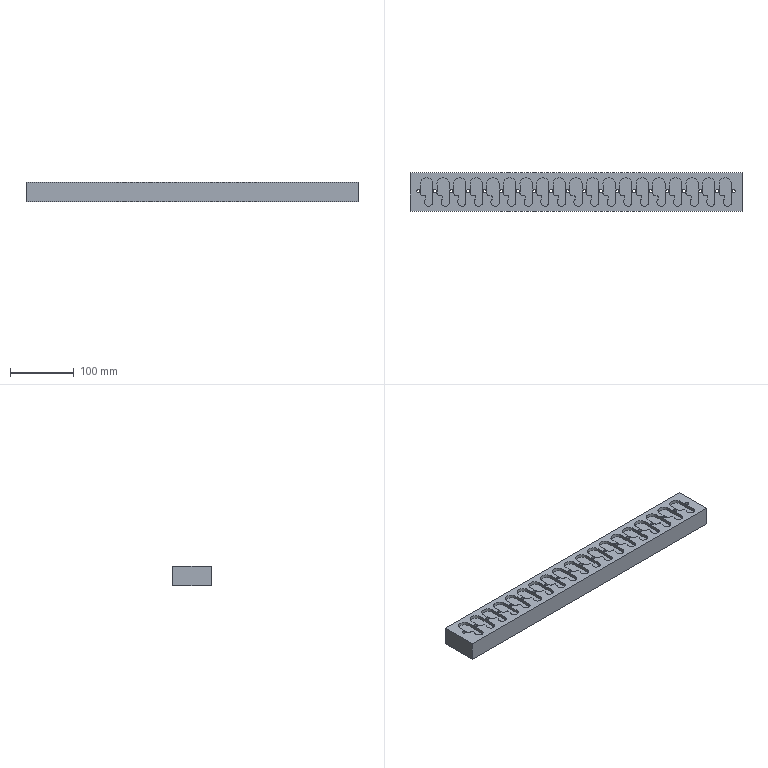CAM job | Mastercam | mm | 3 operations | part box 520 x 60 x 30
1. 2D High Speed (2D Dynamic Mill) | 9 - 7.9 平铣刀
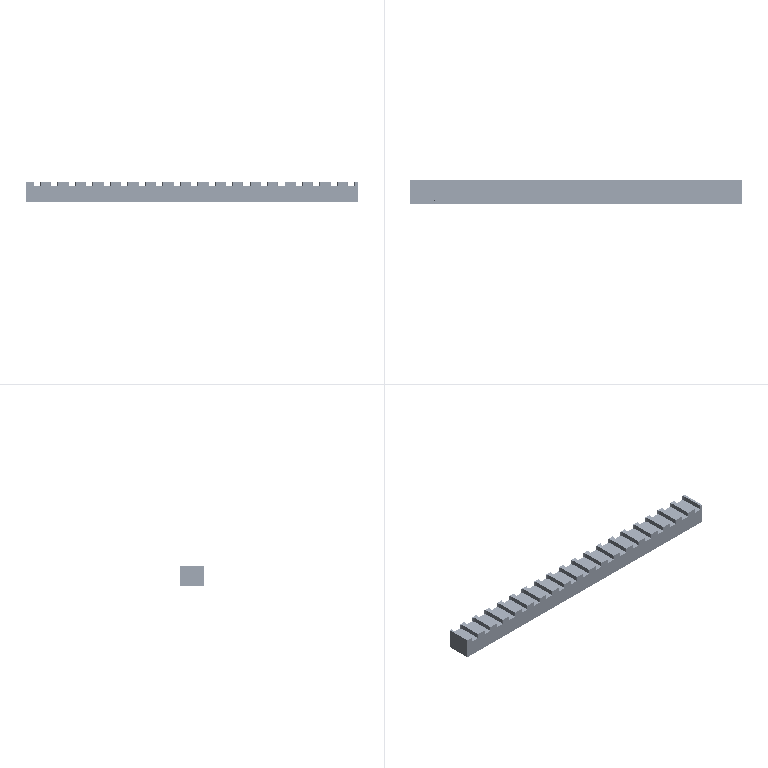2. Drill/Counterbore | 2 - 6 定位钻
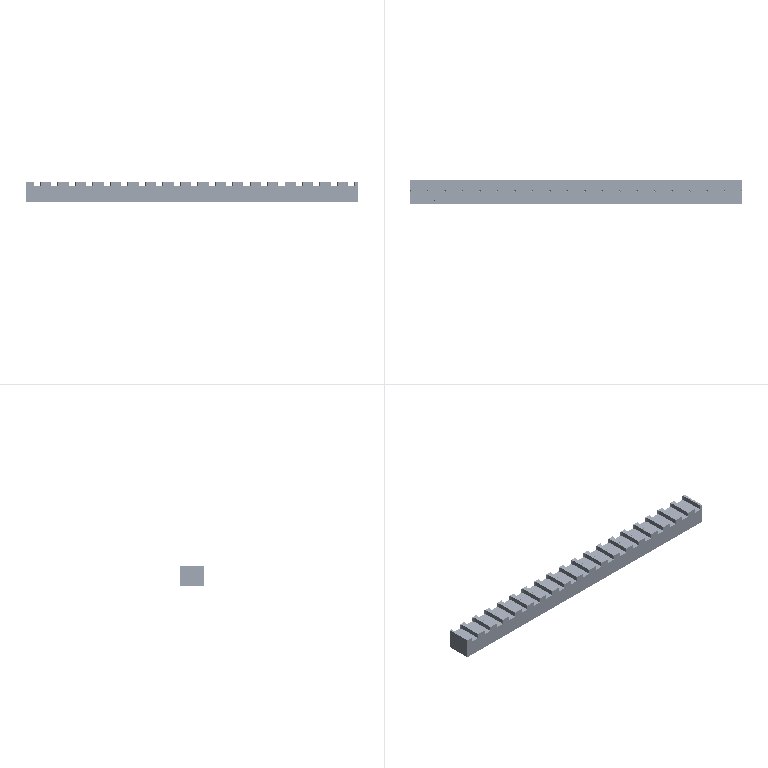3. Peck Drill | 20 - 5.3 钻头